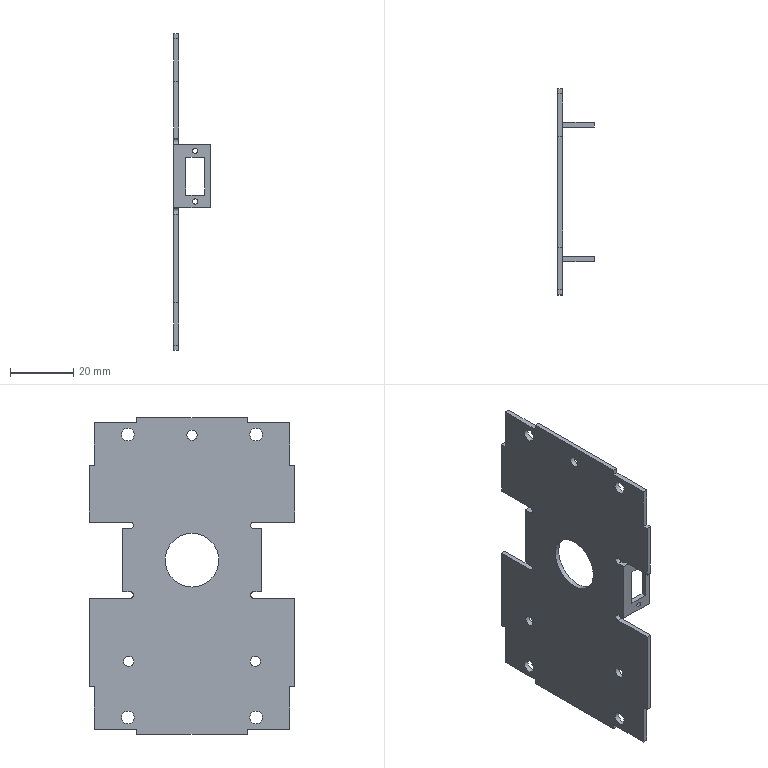Component | NX | COVER | 1 solid | 62 faces | volume 8602 mm3 | plane 46 | cylinder 16 | commonest cylinder face diameters 2 x4 4 x4 1.6 x4 3.2 x3 17 x1